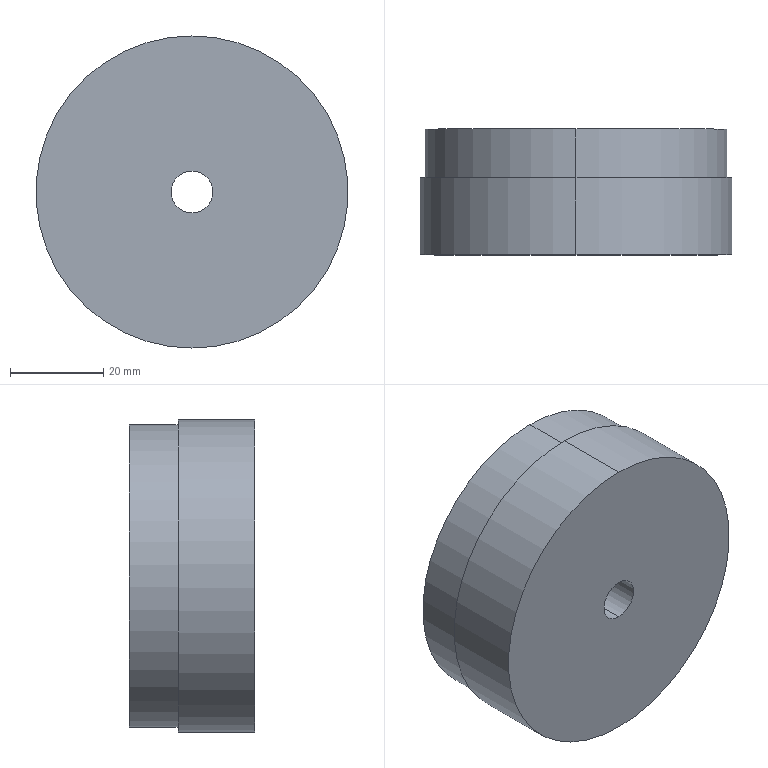Component | SolidWorks | Inline-H010-A_EMSQA30A-A96(0)-1_Inline-H010-2-1 | 1 solid | 58 faces | volume 86334 mm3 | cylinder 27 | cone 16 | plane 15 | commonest cylinder face diameters 4.917 x16 4 x3 67 x2 9 x2 65 x2 32 x2